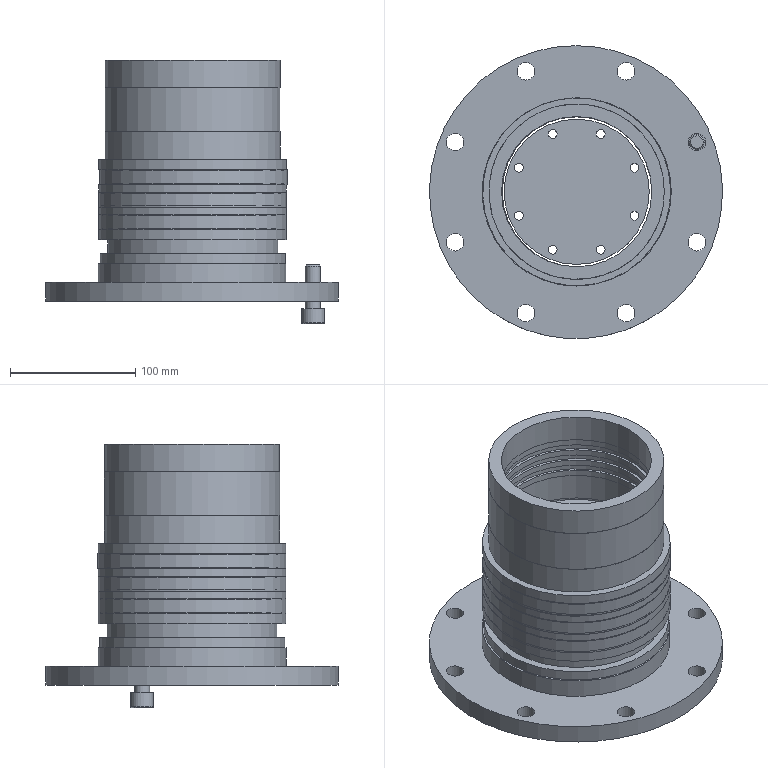Assembly | NX | mm | 14 component files | 14 solids | 179 faces | box 234 x 234 x 210.3 mm | volume 1125108 mm3 | plane 75 | cylinder 68 | cone 29 | torus 7 | commonest cylinder face diameters 132 x9 150 x8 14 x8 7 x8 120 x6 130 x4 140 x3 124 x3
Bill of materials:
CH3404-9 | 2 |  | Thin flat annular ring (washer-like) with plain rectangular cross-section; radial wall width is small relative to diameter.
CH3404-6 | 2 |  | Short cylindrical sleeve or band ring: annulus with axial height noticeably larger than part-1, plain inner and outer cylindrical surfaces.
CH3404-3 | 1 |  | Solid flat circular plate (blind-flange-like disc) with eight evenly spaced through holes on a bolt circle near the outer edge; no central opening.
CH3404-12 | 1 |  | Annular flange plate with a large central bore, eight evenly spaced through holes on a bolt circle, and a raised cylindrical hub/collar on one face; an internal step or ledge is visible inside the bore.
CH3404-10 | 2 |  | Thin flat annular ring with plain rectangular cross-section, similar to part-1 but with a slightly wider radial wall and thinner-looking profile.
CH3404-7 | 1 |  | Tall cylindrical ring/collar with plain outer surface and internal circumferential features (two visible lines/ridges in the bore), possibly an internal thread or grooves.
CH3404-8 | 1 |  | Stepped annular ring with three external diameters: a wide base lip, a middle step and a slightly narrower top band, with a plain cylindrical bore.
GB/T13871-1992 | 3 |  | FB φ150*φ120*12
GB_T70_1_M12X35 | 1 |  | Headed cylindrical pin or bolt-like part: plain cylindrical shank with chamfered free end, and a larger coaxial cylindrical head with a slightly rounded/chamfered bottom edge.
Mates:
1. touch align | CH3404-9 2 face | CH3404-8 1 face
2. touch align | T13871-1992 1 face | CH3404-9 2 face
3. touch align | CH3404-10 1 face | T13871-1992 1 face
4. touch align | T13871-1992 3 face | CH3404-10 1 face
5. touch align | CH3404-10 2 face | T13871-1992 3 face
6. touch align | T13871-1992 2 face | CH3404-10 2 face
7. touch align | CH3404-9 1 face | T13871-1992 2 face
8. touch align | CH3404-7 1 face | CH3404-6 2 face
9. touch align | CH3404-6 1 face | CH3404-7 1 face